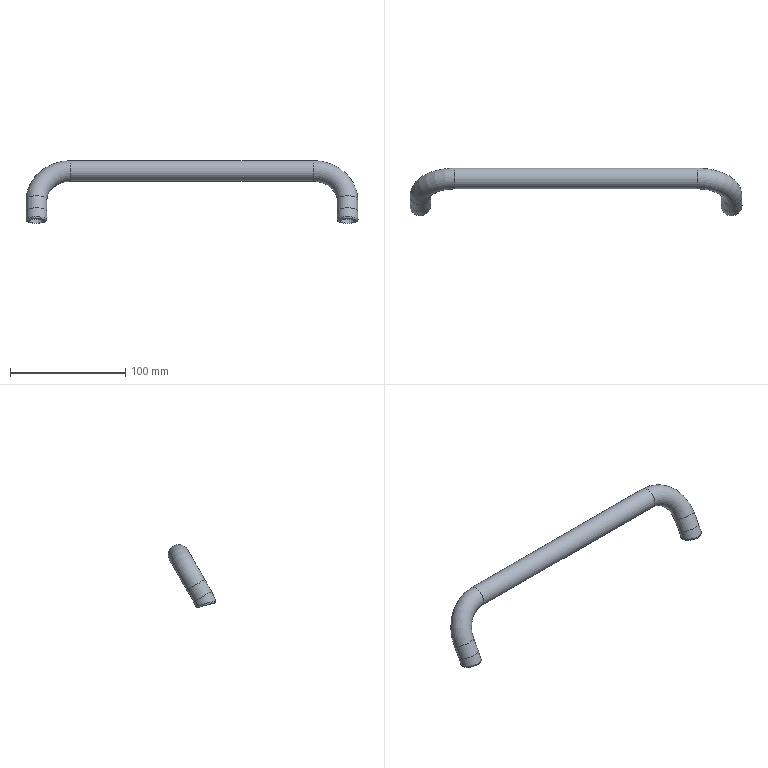Component | NX | FOAM_PAD | 1 solid | 18 faces | box 288 x 41.31 x 54.58 mm | volume 41802 mm3 | torus 8 | cylinder 6 | plane 2 | spline 2 | commonest cylinder face diameters 18 x3 13 x3
STEP:
#1=VALUE_REPRESENTATION_ITEM('',COUNT_MEASURE(0.));
#2=(LENGTH_UNIT()NAMED_UNIT(*)SI_UNIT(.MILLI.,.METRE.));
#3=UNCERTAINTY_MEASURE_WITH_UNIT(LENGTH_MEASURE(0.0508),#2,'','');
#4=(NAMED_UNIT(*)PLANE_ANGLE_UNIT()SI_UNIT($,.RADIAN.));
#5=PLANE_ANGLE_MEASURE_WITH_UNIT(PLANE_ANGLE_MEASURE(0.01745),#4);
#6=DIMENSIONAL_EXPONENTS(0.,0.,0.,0.,0.,0.,0.);
#7=(CONVERSION_BASED_UNIT('',#5)NAMED_UNIT(#6)PLANE_ANGLE_UNIT());
#8=(NAMED_UNIT(*)SI_UNIT($,.STERADIAN.)SOLID_ANGLE_UNIT());
#9=(GEOMETRIC_REPRESENTATION_CONTEXT(3)GLOBAL_UNCERTAINTY_ASSIGNED_CONTEXT((#3))GLOBAL_UNIT_ASSIGNED_CONTEXT((#2,#7,#8))REPRESENTATION_CONTEXT('',''));
#10=REPRESENTATION('',(#1),#9);
#11=VALUE_REPRESENTATION_ITEM('',COUNT_MEASURE(0.));
#12=REPRESENTATION('',(#11),#9);
#13=CARTESIAN_POINT('',(0.,0.,0.));
#14=DIRECTION('',(0.,0.,1.));
#15=DIRECTION('',(1.,0.,0.));
#16=AXIS2_PLACEMENT_3D('',#13,#14,#15);
#17=SHAPE_REPRESENTATION('',(#16),#9);
#18=CARTESIAN_POINT('',(-270.,117.638,-91.446));
#19=VERTEX_POINT('',#18);
#20=CARTESIAN_POINT('',(-272.379,117.638,-91.446));
#21=CARTESIAN_POINT('',(-267.621,117.638,-91.446));
#22=CARTESIAN_POINT('',(-265.309,118.565,-91.699));
#23=CARTESIAN_POINT('',(-261.953,121.809,-92.589));
#24=CARTESIAN_POINT('',(-260.999,124.062,-93.209));
#25=CARTESIAN_POINT('',(-261.001,128.588,-94.462));
#26=CARTESIAN_POINT('',(-261.973,130.853,-95.094));
#27=CARTESIAN_POINT('',(-265.29,134.054,-95.994));
#28=CARTESIAN_POINT('',(-267.615,134.996,-96.263));
#29=CARTESIAN_POINT('',(-272.372,135.,-96.264));
#30=CARTESIAN_POINT('',(-274.703,134.059,-95.996));
#31=CARTESIAN_POINT('',(-278.025,130.858,-95.096));
#32=CARTESIAN_POINT('',(-278.999,128.614,-94.469));
#33=CARTESIAN_POINT('',(-279.001,124.036,-93.202));
#34=CARTESIAN_POINT('',(-278.027,121.79,-92.584));
#35=CARTESIAN_POINT('',(-274.711,118.584,-91.704));
#36=CARTESIAN_POINT('',(-272.379,117.638,-91.446));
#37=CARTESIAN_POINT('',(-267.621,117.638,-91.446));
#38=B_SPLINE_CURVE_WITH_KNOTS('',3,(#20,#21,#22,#23,#24,#25,#26,#27,#28,#29,#30,#31,#32,#33,#34,#35,#36,#37),.UNSPECIFIED.,.T.,.F.,(2,2,2,2,2,2,2,2,2,2,2),(-0.125,0.,0.125,0.25,0.375,0.5,0.625,0.75,0.875,1.,1.125),.UNSPECIFIED.);
#39=EDGE_CURVE('',#19,#19,#38,.T.);
#40=ORIENTED_EDGE('',*,*,#39,.T.);
#41=EDGE_LOOP('',(#40));
#42=FACE_BOUND('',#41,.T.);
#43=CARTESIAN_POINT('',(-270.,121.1,-83.538));
#44=VERTEX_POINT('',#43);
#45=CARTESIAN_POINT('',(-270.,128.894,-88.038));
#46=DIRECTION('',(-0.,-0.5,-0.866));
#47=DIRECTION('',(0.,-0.866,0.5));
#48=AXIS2_PLACEMENT_3D('',#45,#46,#47);
#49=CIRCLE('',#48,9.);
#50=EDGE_CURVE('',#44,#44,#49,.T.);
#51=ORIENTED_EDGE('',*,*,#50,.T.);
#52=EDGE_LOOP('',(#51));
#53=FACE_BOUND('',#52,.T.);
#54=CARTESIAN_POINT('',(-270.,154.875,-103.038));
#55=DIRECTION('',(1.,0.,0.));
#56=DIRECTION('',(0.,0.,-1.));
#57=AXIS2_PLACEMENT_3D('',#54,#55,#56);
#58=TOROIDAL_SURFACE('',#57,30.,9.);
#59=ADVANCED_FACE('',(#42,#53),#58,.T.);
#60=CARTESIAN_POINT('',(-270.,123.265,-84.788));
#61=VERTEX_POINT('',#60);
#62=CARTESIAN_POINT('',(-270.,128.894,-88.038));
#63=DIRECTION('',(-0.,-0.5,-0.866));
#64=DIRECTION('',(0.,-0.866,0.5));
#65=AXIS2_PLACEMENT_3D('',#62,#63,#64);
#66=CIRCLE('',#65,6.5);
#67=EDGE_CURVE('',#61,#61,#66,.T.);
#68=ORIENTED_EDGE('',*,*,#67,.F.);
#69=EDGE_LOOP('',(#68));
#70=FACE_BOUND('',#69,.T.);
#71=CARTESIAN_POINT('',(-270.,119.619,-93.592));
#72=VERTEX_POINT('',#71);
#73=CARTESIAN_POINT('',(-270.,125.897,-95.274));
#74=DIRECTION('',(-0.,-0.2588,-0.9659));
#75=DIRECTION('',(0.,-0.9659,0.2588));
#76=AXIS2_PLACEMENT_3D('',#73,#74,#75);
#77=CIRCLE('',#76,6.5);
#78=EDGE_CURVE('',#72,#72,#77,.T.);
#79=ORIENTED_EDGE('',*,*,#78,.T.);
#80=EDGE_LOOP('',(#79));
#81=FACE_BOUND('',#80,.T.);
#82=CARTESIAN_POINT('',(-270.,154.875,-103.038));
#83=DIRECTION('',(1.,0.,0.));
#84=DIRECTION('',(0.,0.,-1.));
#85=AXIS2_PLACEMENT_3D('',#82,#83,#84);
#86=TOROIDAL_SURFACE('',#85,30.,6.5);
#87=ADVANCED_FACE('',(#70,#81),#86,.F.);
#88=CARTESIAN_POINT('',(-270.,127.081,-73.179));
#89=VERTEX_POINT('',#88);
#90=CARTESIAN_POINT('',(-270.,134.875,-77.679));
#91=DIRECTION('',(-0.,-0.5,-0.866));
#92=DIRECTION('',(0.,-0.866,0.5));
#93=AXIS2_PLACEMENT_3D('',#90,#91,#92);
#94=CIRCLE('',#93,9.);
#95=EDGE_CURVE('',#89,#89,#94,.T.);
#96=ORIENTED_EDGE('',*,*,#95,.T.);
#97=EDGE_LOOP('',(#96));
#98=FACE_BOUND('',#97,.T.);
#99=ORIENTED_EDGE('',*,*,#50,.F.);
#100=EDGE_LOOP('',(#99));
#101=FACE_BOUND('',#100,.T.);
#102=CARTESIAN_POINT('',(-270.,134.875,-77.679));
#103=DIRECTION('',(0.,-0.5,-0.866));
#104=DIRECTION('',(0.,0.866,-0.5));
#105=AXIS2_PLACEMENT_3D('',#102,#103,#104);
#106=CYLINDRICAL_SURFACE('',#105,9.);
#107=ADVANCED_FACE('',(#98,#101),#106,.T.);
#108=CARTESIAN_POINT('',(-270.,129.246,-74.429));
#109=VERTEX_POINT('',#108);
#110=CARTESIAN_POINT('',(-270.,134.875,-77.679));
#111=DIRECTION('',(-0.,-0.5,-0.866));
#112=DIRECTION('',(0.,-0.866,0.5));
#113=AXIS2_PLACEMENT_3D('',#110,#111,#112);
#114=CIRCLE('',#113,6.5);
#115=EDGE_CURVE('',#109,#109,#114,.T.);
#116=ORIENTED_EDGE('',*,*,#115,.F.);
#117=EDGE_LOOP('',(#116));
#118=FACE_BOUND('',#117,.T.);
#119=ORIENTED_EDGE('',*,*,#67,.T.);
#120=EDGE_LOOP('',(#119));
#121=FACE_BOUND('',#120,.T.);
#122=CARTESIAN_POINT('',(-270.,134.875,-77.679));
#123=DIRECTION('',(0.,-0.5,-0.866));
#124=DIRECTION('',(0.,0.866,-0.5));
#125=AXIS2_PLACEMENT_3D('',#122,#123,#124);
#126=CYLINDRICAL_SURFACE('',#125,6.5);
#127=ADVANCED_FACE('',(#118,#121),#126,.F.);
#128=CARTESIAN_POINT('',(-240.,142.081,-47.199));
#129=VERTEX_POINT('',#128);
#130=CARTESIAN_POINT('',(-240.,149.875,-51.699));
#131=DIRECTION('',(-1.,-0.,0.));
#132=DIRECTION('',(0.,-0.866,0.5));
#133=AXIS2_PLACEMENT_3D('',#130,#131,#132);
#134=CIRCLE('',#133,9.);
#135=EDGE_CURVE('',#129,#129,#134,.T.);
#136=ORIENTED_EDGE('',*,*,#135,.T.);
#137=EDGE_LOOP('',(#136));
#138=FACE_BOUND('',#137,.T.);
#139=ORIENTED_EDGE('',*,*,#95,.F.);
#140=EDGE_LOOP('',(#139));
#141=FACE_BOUND('',#140,.T.);
#142=CARTESIAN_POINT('',(-240.,134.875,-77.679));
#143=DIRECTION('',(0.,-0.866,0.5));
#144=DIRECTION('',(0.,-0.5,-0.866));
#145=AXIS2_PLACEMENT_3D('',#142,#143,#144);
#146=TOROIDAL_SURFACE('',#145,30.,9.);
#147=ADVANCED_FACE('',(#138,#141),#146,.T.);
#148=CARTESIAN_POINT('',(-240.,144.246,-48.449));
#149=VERTEX_POINT('',#148);
#150=CARTESIAN_POINT('',(-240.,149.875,-51.699));
#151=DIRECTION('',(-1.,-0.,0.));
#152=DIRECTION('',(0.,-0.866,0.5));
#153=AXIS2_PLACEMENT_3D('',#150,#151,#152);
#154=CIRCLE('',#153,6.5);
#155=EDGE_CURVE('',#149,#149,#154,.T.);
#156=ORIENTED_EDGE('',*,*,#155,.F.);
#157=EDGE_LOOP('',(#156));
#158=FACE_BOUND('',#157,.T.);
#159=ORIENTED_EDGE('',*,*,#115,.T.);
#160=EDGE_LOOP('',(#159));
#161=FACE_BOUND('',#160,.T.);
#162=CARTESIAN_POINT('',(-240.,134.875,-77.679));
#163=DIRECTION('',(0.,-0.866,0.5));
#164=DIRECTION('',(0.,-0.5,-0.866));
#165=AXIS2_PLACEMENT_3D('',#162,#163,#164);
#166=TOROIDAL_SURFACE('',#165,30.,6.5);
#167=ADVANCED_FACE('',(#158,#161),#166,.F.);
#168=CARTESIAN_POINT('',(-30.,142.081,-47.199));
#169=VERTEX_POINT('',#168);
#170=CARTESIAN_POINT('',(-30.,149.875,-51.699));
#171=DIRECTION('',(-1.,-0.,0.));
#172=DIRECTION('',(0.,-0.866,0.5));
#173=AXIS2_PLACEMENT_3D('',#170,#171,#172);
#174=CIRCLE('',#173,9.);
#175=EDGE_CURVE('',#169,#169,#174,.T.);
#176=ORIENTED_EDGE('',*,*,#175,.T.);
#177=EDGE_LOOP('',(#176));
#178=FACE_BOUND('',#177,.T.);
#179=ORIENTED_EDGE('',*,*,#135,.F.);
#180=EDGE_LOOP('',(#179));
#181=FACE_BOUND('',#180,.T.);
#182=CARTESIAN_POINT('',(-30.,149.875,-51.699));
#183=DIRECTION('',(-1.,0.,0.));
#184=DIRECTION('',(0.,0.,1.));
#185=AXIS2_PLACEMENT_3D('',#182,#183,#184);
#186=CYLINDRICAL_SURFACE('',#185,9.);
#187=ADVANCED_FACE('',(#178,#181),#186,.T.);
#188=CARTESIAN_POINT('',(-30.,144.246,-48.449));
#189=VERTEX_POINT('',#188);
#190=CARTESIAN_POINT('',(-30.,149.875,-51.699));
#191=DIRECTION('',(-1.,-0.,0.));
#192=DIRECTION('',(0.,-0.866,0.5));
#193=AXIS2_PLACEMENT_3D('',#190,#191,#192);
#194=CIRCLE('',#193,6.5);
#195=EDGE_CURVE('',#189,#189,#194,.T.);
#196=ORIENTED_EDGE('',*,*,#195,.F.);
#197=EDGE_LOOP('',(#196));
#198=FACE_BOUND('',#197,.T.);
#199=ORIENTED_EDGE('',*,*,#155,.T.);
#200=EDGE_LOOP('',(#199));
#201=FACE_BOUND('',#200,.T.);
#202=CARTESIAN_POINT('',(-30.,149.875,-51.699));
#203=DIRECTION('',(-1.,0.,0.));
#204=DIRECTION('',(0.,0.,1.));
#205=AXIS2_PLACEMENT_3D('',#202,#203,#204);
#206=CYLINDRICAL_SURFACE('',#205,6.5);
#207=ADVANCED_FACE('',(#198,#201),#206,.F.);
#208=CARTESIAN_POINT('',(-0.,127.081,-73.179));
#209=VERTEX_POINT('',#208);
#210=CARTESIAN_POINT('',(-0.,134.875,-77.679));
#211=DIRECTION('',(0.,0.5,0.866));
#212=DIRECTION('',(0.,-0.866,0.5));
#213=AXIS2_PLACEMENT_3D('',#210,#211,#212);
#214=CIRCLE('',#213,9.);
#215=EDGE_CURVE('',#209,#209,#214,.T.);
#216=ORIENTED_EDGE('',*,*,#215,.T.);
#217=EDGE_LOOP('',(#216));
#218=FACE_BOUND('',#217,.T.);
#219=ORIENTED_EDGE('',*,*,#175,.F.);
#220=EDGE_LOOP('',(#219));
#221=FACE_BOUND('',#220,.T.);
#222=CARTESIAN_POINT('',(-30.,134.875,-77.679));
#223=DIRECTION('',(0.,-0.866,0.5));
#224=DIRECTION('',(0.,-0.5,-0.866));
#225=AXIS2_PLACEMENT_3D('',#222,#223,#224);
#226=TOROIDAL_SURFACE('',#225,30.,9.);
#227=ADVANCED_FACE('',(#218,#221),#226,.T.);
#228=CARTESIAN_POINT('',(-0.,129.246,-74.429));
#229=VERTEX_POINT('',#228);
#230=CARTESIAN_POINT('',(-0.,134.875,-77.679));
#231=DIRECTION('',(0.,0.5,0.866));
#232=DIRECTION('',(0.,-0.866,0.5));
#233=AXIS2_PLACEMENT_3D('',#230,#231,#232);
#234=CIRCLE('',#233,6.5);
#235=EDGE_CURVE('',#229,#229,#234,.T.);
#236=ORIENTED_EDGE('',*,*,#235,.F.);
#237=EDGE_LOOP('',(#236));
#238=FACE_BOUND('',#237,.T.);
#239=ORIENTED_EDGE('',*,*,#195,.T.);
#240=EDGE_LOOP('',(#239));
#241=FACE_BOUND('',#240,.T.);
#242=CARTESIAN_POINT('',(-30.,134.875,-77.679));
#243=DIRECTION('',(0.,-0.866,0.5));
#244=DIRECTION('',(0.,-0.5,-0.866));
#245=AXIS2_PLACEMENT_3D('',#242,#243,#244);
#246=TOROIDAL_SURFACE('',#245,30.,6.5);
#247=ADVANCED_FACE('',(#238,#241),#246,.F.);
#248=CARTESIAN_POINT('',(-0.,121.1,-83.538));
#249=VERTEX_POINT('',#248);
#250=CARTESIAN_POINT('',(-0.,128.894,-88.038));
#251=DIRECTION('',(0.,0.5,0.866));
#252=DIRECTION('',(0.,-0.866,0.5));
#253=AXIS2_PLACEMENT_3D('',#250,#251,#252);
#254=CIRCLE('',#253,9.);
#255=EDGE_CURVE('',#249,#249,#254,.T.);
#256=ORIENTED_EDGE('',*,*,#255,.T.);
#257=EDGE_LOOP('',(#256));
#258=FACE_BOUND('',#257,.T.);
#259=ORIENTED_EDGE('',*,*,#215,.F.);
#260=EDGE_LOOP('',(#259));
#261=FACE_BOUND('',#260,.T.);
#262=CARTESIAN_POINT('',(-0.,128.894,-88.038));
#263=DIRECTION('',(0.,0.5,0.866));
#264=DIRECTION('',(0.,-0.866,0.5));
#265=AXIS2_PLACEMENT_3D('',#262,#263,#264);
#266=CYLINDRICAL_SURFACE('',#265,9.);
#267=ADVANCED_FACE('',(#258,#261),#266,.T.);
#268=CARTESIAN_POINT('',(-0.,123.265,-84.788));
#269=VERTEX_POINT('',#268);
#270=CARTESIAN_POINT('',(-0.,128.894,-88.038));
#271=DIRECTION('',(0.,0.5,0.866));
#272=DIRECTION('',(0.,-0.866,0.5));
#273=AXIS2_PLACEMENT_3D('',#270,#271,#272);
#274=CIRCLE('',#273,6.5);
#275=EDGE_CURVE('',#269,#269,#274,.T.);
#276=ORIENTED_EDGE('',*,*,#275,.F.);
#277=EDGE_LOOP('',(#276));
#278=FACE_BOUND('',#277,.T.);
#279=ORIENTED_EDGE('',*,*,#235,.T.);
#280=EDGE_LOOP('',(#279));
#281=FACE_BOUND('',#280,.T.);
#282=CARTESIAN_POINT('',(-0.,128.894,-88.038));
#283=DIRECTION('',(0.,0.5,0.866));
#284=DIRECTION('',(0.,-0.866,0.5));
#285=AXIS2_PLACEMENT_3D('',#282,#283,#284);
#286=CYLINDRICAL_SURFACE('',#285,6.5);
#287=ADVANCED_FACE('',(#278,#281),#286,.F.);
#288=ORIENTED_EDGE('',*,*,#275,.T.);
#289=EDGE_LOOP('',(#288));
#290=FACE_BOUND('',#289,.T.);
#291=CARTESIAN_POINT('',(-0.,119.619,-93.592));
#292=VERTEX_POINT('',#291);
#293=CARTESIAN_POINT('',(-0.,125.897,-95.274));
#294=DIRECTION('',(0.,0.2588,0.9659));
#295=DIRECTION('',(0.,-0.9659,0.2588));
#296=AXIS2_PLACEMENT_3D('',#293,#294,#295);
#297=CIRCLE('',#296,6.5);
#298=EDGE_CURVE('',#292,#292,#297,.T.);
#299=ORIENTED_EDGE('',*,*,#298,.F.);
#300=EDGE_LOOP('',(#299));
#301=FACE_BOUND('',#300,.T.);
#302=CARTESIAN_POINT('',(-0.,154.875,-103.038));
#303=DIRECTION('',(1.,0.,0.));
#304=DIRECTION('',(0.,0.,-1.));
#305=AXIS2_PLACEMENT_3D('',#302,#303,#304);
#306=TOROIDAL_SURFACE('',#305,30.,6.5);
#307=ADVANCED_FACE('',(#290,#301),#306,.F.);
#308=CARTESIAN_POINT('',(-0.,117.638,-91.446));
#309=VERTEX_POINT('',#308);
#310=CARTESIAN_POINT('',(-2.379,117.638,-91.446));
#311=CARTESIAN_POINT('',(2.379,117.638,-91.446));
#312=CARTESIAN_POINT('',(4.711,118.584,-91.704));
#313=CARTESIAN_POINT('',(8.027,121.79,-92.584));
#314=CARTESIAN_POINT('',(9.001,124.036,-93.202));
#315=CARTESIAN_POINT('',(8.999,128.614,-94.469));
#316=CARTESIAN_POINT('',(8.025,130.858,-95.096));
#317=CARTESIAN_POINT('',(4.703,134.059,-95.996));
#318=CARTESIAN_POINT('',(2.372,135.,-96.264));
#319=CARTESIAN_POINT('',(-2.385,134.996,-96.263));
#320=CARTESIAN_POINT('',(-4.71,134.054,-95.994));
#321=CARTESIAN_POINT('',(-8.027,130.853,-95.094));
#322=CARTESIAN_POINT('',(-8.999,128.588,-94.462));
#323=CARTESIAN_POINT('',(-9.001,124.062,-93.209));
#324=CARTESIAN_POINT('',(-8.047,121.809,-92.589));
#325=CARTESIAN_POINT('',(-4.691,118.565,-91.699));
#326=CARTESIAN_POINT('',(-2.379,117.638,-91.446));
#327=CARTESIAN_POINT('',(2.379,117.638,-91.446));
#328=B_SPLINE_CURVE_WITH_KNOTS('',3,(#310,#311,#312,#313,#314,#315,#316,#317,#318,#319,#320,#321,#322,#323,#324,#325,#326,#327),.UNSPECIFIED.,.T.,.F.,(2,2,2,2,2,2,2,2,2,2,2),(-0.125,0.,0.125,0.25,0.375,0.5,0.625,0.75,0.875,1.,1.125),.UNSPECIFIED.);
#329=EDGE_CURVE('',#309,#309,#328,.T.);
#330=ORIENTED_EDGE('',*,*,#329,.T.);
#331=EDGE_LOOP('',(#330));
#332=FACE_BOUND('',#331,.T.);
#333=ORIENTED_EDGE('',*,*,#255,.F.);
#334=EDGE_LOOP('',(#333));
#335=FACE_BOUND('',#334,.T.);
#336=CARTESIAN_POINT('',(-0.,154.875,-103.038));
#337=DIRECTION('',(1.,0.,0.));
#338=DIRECTION('',(0.,0.,-1.));
#339=AXIS2_PLACEMENT_3D('',#336,#337,#338);
#340=TOROIDAL_SURFACE('',#339,30.,9.);
#341=ADVANCED_FACE('',(#332,#335),#340,.T.);
#342=CARTESIAN_POINT('',(-270.,118.682,-93.341));
#343=VERTEX_POINT('',#342);
#344=CARTESIAN_POINT('',(-268.017,118.682,-93.341));
#345=CARTESIAN_POINT('',(-271.983,118.682,-93.341));
#346=CARTESIAN_POINT('',(-273.927,119.472,-93.552));
#347=CARTESIAN_POINT('',(-276.69,122.149,-94.269));
#348=CARTESIAN_POINT('',(-277.501,124.025,-94.772));
#349=CARTESIAN_POINT('',(-277.499,127.849,-95.797));
#350=CARTESIAN_POINT('',(-276.687,129.725,-96.299));
#351=CARTESIAN_POINT('',(-273.919,132.403,-97.017));
#352=CARTESIAN_POINT('',(-271.977,133.192,-97.228));
#353=CARTESIAN_POINT('',(-268.012,133.189,-97.228));
#354=CARTESIAN_POINT('',(-266.074,132.399,-97.016));
#355=CARTESIAN_POINT('',(-263.311,129.72,-96.298));
#356=CARTESIAN_POINT('',(-262.501,127.828,-95.791));
#357=CARTESIAN_POINT('',(-262.499,124.047,-94.778));
#358=CARTESIAN_POINT('',(-263.293,122.165,-94.274));
#359=CARTESIAN_POINT('',(-266.09,119.456,-93.548));
#360=CARTESIAN_POINT('',(-268.017,118.682,-93.341));
#361=CARTESIAN_POINT('',(-271.983,118.682,-93.341));
#362=B_SPLINE_CURVE_WITH_KNOTS('',3,(#344,#345,#346,#347,#348,#349,#350,#351,#352,#353,#354,#355,#356,#357,#358,#359,#360,#361),.UNSPECIFIED.,.T.,.F.,(2,2,2,2,2,2,2,2,2,2,2),(-0.125,0.,0.125,0.25,0.375,0.5,0.625,0.75,0.875,1.,1.125),.UNSPECIFIED.);
#363=EDGE_CURVE('',#343,#343,#362,.T.);
#364=ORIENTED_EDGE('',*,*,#363,.T.);
#365=EDGE_LOOP('',(#364));
#366=FACE_BOUND('',#365,.T.);
#367=ORIENTED_EDGE('',*,*,#78,.F.);
#368=EDGE_LOOP('',(#367));
#369=FACE_BOUND('',#368,.T.);
#370=CARTESIAN_POINT('',(-270.,125.897,-95.274));
#371=DIRECTION('',(-0.,-0.2588,-0.9659));
#372=DIRECTION('',(0.,-0.9659,0.2588));
#373=AXIS2_PLACEMENT_3D('',#370,#371,#372);
#374=PLANE('',#373);
#375=ADVANCED_FACE('',(#366,#369),#374,.T.);
#376=CARTESIAN_POINT('',(-0.,118.682,-93.341));
#377=VERTEX_POINT('',#376);
#378=CARTESIAN_POINT('',(1.983,118.682,-93.341));
#379=CARTESIAN_POINT('',(-1.983,118.682,-93.341));
#380=CARTESIAN_POINT('',(-3.91,119.456,-93.548));
#381=CARTESIAN_POINT('',(-6.707,122.165,-94.274));
#382=CARTESIAN_POINT('',(-7.501,124.047,-94.778));
#383=CARTESIAN_POINT('',(-7.499,127.828,-95.791));
#384=CARTESIAN_POINT('',(-6.689,129.72,-96.298));
#385=CARTESIAN_POINT('',(-3.926,132.399,-97.016));
#386=CARTESIAN_POINT('',(-1.988,133.189,-97.228));
#387=CARTESIAN_POINT('',(1.977,133.192,-97.228));
#388=CARTESIAN_POINT('',(3.92,132.403,-97.017));
#389=CARTESIAN_POINT('',(6.687,129.725,-96.299));
#390=CARTESIAN_POINT('',(7.499,127.849,-95.797));
#391=CARTESIAN_POINT('',(7.501,124.025,-94.772));
#392=CARTESIAN_POINT('',(6.69,122.149,-94.269));
#393=CARTESIAN_POINT('',(3.927,119.472,-93.552));
#394=CARTESIAN_POINT('',(1.983,118.682,-93.341));
#395=CARTESIAN_POINT('',(-1.983,118.682,-93.341));
#396=B_SPLINE_CURVE_WITH_KNOTS('',3,(#378,#379,#380,#381,#382,#383,#384,#385,#386,#387,#388,#389,#390,#391,#392,#393,#394,#395),.UNSPECIFIED.,.T.,.F.,(2,2,2,2,2,2,2,2,2,2,2),(-0.125,0.,0.125,0.25,0.375,0.5,0.625,0.75,0.875,1.,1.125),.UNSPECIFIED.);
#397=EDGE_CURVE('',#377,#377,#396,.T.);
#398=ORIENTED_EDGE('',*,*,#397,.T.);
#399=EDGE_LOOP('',(#398));
#400=FACE_BOUND('',#399,.T.);
#401=ORIENTED_EDGE('',*,*,#298,.T.);
#402=EDGE_LOOP('',(#401));
#403=FACE_BOUND('',#402,.T.);
#404=CARTESIAN_POINT('',(-0.,125.897,-95.274));
#405=DIRECTION('',(0.,0.2588,0.9659));
#406=DIRECTION('',(0.,-0.9659,0.2588));
#407=AXIS2_PLACEMENT_3D('',#404,#405,#406);
#408=PLANE('',#407);
#409=ADVANCED_FACE('',(#400,#403),#408,.F.);
#410=ORIENTED_EDGE('',*,*,#39,.F.);
#411=EDGE_LOOP('',(#410));
#412=FACE_BOUND('',#411,.T.);
#413=ORIENTED_EDGE('',*,*,#363,.F.);
#414=EDGE_LOOP('',(#413));
#415=FACE_BOUND('',#414,.T.);
#416=CARTESIAN_POINT('',(-269.053,117.686,-91.459));
#417=CARTESIAN_POINT('',(-269.047,117.223,-92.95));
#418=CARTESIAN_POINT('',(-269.211,118.722,-93.351));
#419=CARTESIAN_POINT('',(-270.237,117.565,-91.426));
#420=CARTESIAN_POINT('',(-270.239,117.1,-92.917));
#421=CARTESIAN_POINT('',(-270.197,118.621,-93.324));
#422=CARTESIAN_POINT('',(-271.423,117.672,-91.455));
#423=CARTESIAN_POINT('',(-271.432,117.208,-92.946));
#424=CARTESIAN_POINT('',(-271.186,118.71,-93.348));
#425=CARTESIAN_POINT('',(-273.687,118.319,-91.632));
#426=CARTESIAN_POINT('',(-273.71,117.864,-93.121));
#427=CARTESIAN_POINT('',(-273.072,119.25,-93.493));
#428=CARTESIAN_POINT('',(-274.75,118.86,-91.78));
#429=CARTESIAN_POINT('',(-274.778,118.411,-93.268));
#430=CARTESIAN_POINT('',(-273.959,119.702,-93.614));
#431=CARTESIAN_POINT('',(-277.489,120.999,-92.367));
#432=CARTESIAN_POINT('',(-277.52,120.574,-93.847));
#433=CARTESIAN_POINT('',(-276.241,121.488,-94.092));
#434=CARTESIAN_POINT('',(-278.703,123.156,-92.959));
#435=CARTESIAN_POINT('',(-278.727,122.742,-94.429));
#436=CARTESIAN_POINT('',(-277.252,123.289,-94.575));
#437=CARTESIAN_POINT('',(-279.074,126.533,-93.893));
#438=CARTESIAN_POINT('',(-279.072,126.143,-95.34));
#439=CARTESIAN_POINT('',(-277.561,126.11,-95.331));
#440=CARTESIAN_POINT('',(-278.966,127.687,-94.213));
#441=CARTESIAN_POINT('',(-278.955,127.298,-95.649));
#442=CARTESIAN_POINT('',(-277.471,127.074,-95.589));
#443=CARTESIAN_POINT('',(-278.299,129.867,-94.82));
#444=CARTESIAN_POINT('',(-278.269,129.472,-96.232));
#445=CARTESIAN_POINT('',(-276.916,128.897,-96.078));
#446=CARTESIAN_POINT('',(-277.748,130.884,-95.104));
#447=CARTESIAN_POINT('',(-277.712,130.483,-96.503));
#448=CARTESIAN_POINT('',(-276.456,129.747,-96.306));
#449=CARTESIAN_POINT('',(-275.509,133.556,-95.853));
#450=CARTESIAN_POINT('',(-275.471,133.12,-97.209));
#451=CARTESIAN_POINT('',(-274.591,131.982,-96.904));
#452=CARTESIAN_POINT('',(-273.3,134.71,-96.181));
#453=CARTESIAN_POINT('',(-273.269,134.263,-97.515));
#454=CARTESIAN_POINT('',(-272.75,132.949,-97.163));
#455=CARTESIAN_POINT('',(-268.593,135.19,-96.317));
#456=CARTESIAN_POINT('',(-268.61,134.733,-97.641));
#457=CARTESIAN_POINT('',(-268.827,133.351,-97.271));
#458=CARTESIAN_POINT('',(-266.18,134.505,-96.122));
#459=CARTESIAN_POINT('',(-266.209,134.056,-97.46));
#460=CARTESIAN_POINT('',(-266.817,132.777,-97.117));
#461=CARTESIAN_POINT('',(-263.412,132.344,-95.513));
#462=CARTESIAN_POINT('',(-263.454,131.93,-96.89));
#463=CARTESIAN_POINT('',(-264.51,130.968,-96.633));
#464=CARTESIAN_POINT('',(-262.652,131.46,-95.265));
#465=CARTESIAN_POINT('',(-262.691,131.054,-96.656));
#466=CARTESIAN_POINT('',(-263.876,130.229,-96.434));
#467=CARTESIAN_POINT('',(-261.528,129.463,-94.707));
#468=CARTESIAN_POINT('',(-261.554,129.07,-96.124));
#469=CARTESIAN_POINT('',(-262.94,128.559,-95.987));
#470=CARTESIAN_POINT('',(-261.172,128.356,-94.399));
#471=CARTESIAN_POINT('',(-261.19,127.966,-95.828));
#472=CARTESIAN_POINT('',(-262.644,127.633,-95.739));
#473=CARTESIAN_POINT('',(-260.804,124.98,-93.462));
#474=CARTESIAN_POINT('',(-260.79,124.577,-94.92));
#475=CARTESIAN_POINT('',(-262.337,124.813,-94.983));
#476=CARTESIAN_POINT('',(-261.524,122.627,-92.814));
#477=CARTESIAN_POINT('',(-261.499,122.215,-94.287));
#478=CARTESIAN_POINT('',(-262.936,122.847,-94.457));
#479=CARTESIAN_POINT('',(-263.738,119.983,-92.088));
#480=CARTESIAN_POINT('',(-263.705,119.548,-93.573));
#481=CARTESIAN_POINT('',(-264.781,120.64,-93.865));
#482=CARTESIAN_POINT('',(-264.66,119.24,-91.884));
#483=CARTESIAN_POINT('',(-264.63,118.796,-93.371));
#484=CARTESIAN_POINT('',(-265.55,120.019,-93.699));
#485=CARTESIAN_POINT('',(-266.734,118.15,-91.586));
#486=CARTESIAN_POINT('',(-266.713,117.693,-93.076));
#487=CARTESIAN_POINT('',(-267.278,119.11,-93.455));
#488=CARTESIAN_POINT('',(-267.87,117.807,-91.492));
#489=CARTESIAN_POINT('',(-267.856,117.345,-92.982));
#490=CARTESIAN_POINT('',(-268.225,118.823,-93.378));
#491=CARTESIAN_POINT('',(-269.053,117.686,-91.459));
#492=CARTESIAN_POINT('',(-269.047,117.223,-92.95));
#493=CARTESIAN_POINT('',(-269.211,118.722,-93.351));
#494=(BOUNDED_SURFACE()B_SPLINE_SURFACE(3,2,((#416,#417,#418),(#419,#420,#421),(#422,#423,#424),(#425,#426,#427),(#428,#429,#430),(#431,#432,#433),(#434,#435,#436),(#437,#438,#439),(#440,#441,#442),(#443,#444,#445),(#446,#447,#448),(#449,#450,#451),(#452,#453,#454),(#455,#456,#457),(#458,#459,#460),(#461,#462,#463),(#464,#465,#466),(#467,#468,#469),(#470,#471,#472),(#473,#474,#475),(#476,#477,#478),(#479,#480,#481),(#482,#483,#484),(#485,#486,#487),(#488,#489,#490),(#491,#492,#493)),.UNSPECIFIED.,.T.,.F.,.F.)B_SPLINE_SURFACE_WITH_KNOTS((1,3,2,2,2,2,2,2,2,2,2,2,2,3,1),(3,3),(-0.0625,0.,0.0625,0.125,0.25,0.3125,0.375,0.5,0.625,0.6875,0.75,0.875,0.9375,1.,1.062),(0.,1.),.UNSPECIFIED.)GEOMETRIC_REPRESENTATION_ITEM()RATIONAL_B_SPLINE_SURFACE(((1.,0.6929,1.),(1.,0.6927,1.),(1.,0.6929,1.),(1.,0.6937,1.),(1.,0.6945,1.),(1.,0.6976,1.),(1.,0.7009,1.),(1.,0.7075,1.),(1.,0.7099,1.),(1.,0.715,1.),(1.,0.7177,1.),(1.,0.7252,1.),(1.,0.7293,1.),(1.,0.731,1.),(1.,0.7284,1.),(1.,0.7217,1.),(1.,0.7192,1.),(1.,0.714,1.),(1.,0.7114,1.),(1.,0.7042,1.),(1.,0.7002,1.),(1.,0.6961,1.),(1.,0.695,1.),(1.,0.6935,1.),(1.,0.693,1.),(1.,0.6929,1.)))REPRESENTATION_ITEM('')SURFACE());
#495=ADVANCED_FACE('',(#412,#415),#494,.T.);
#496=ORIENTED_EDGE('',*,*,#397,.F.);
#497=EDGE_LOOP('',(#496));
#498=FACE_BOUND('',#497,.T.);
#499=ORIENTED_EDGE('',*,*,#329,.F.);
#500=EDGE_LOOP('',(#499));
#501=FACE_BOUND('',#500,.T.);
#502=CARTESIAN_POINT('',(-0.7888,118.722,-93.351));
#503=CARTESIAN_POINT('',(-0.9531,117.223,-92.95));
#504=CARTESIAN_POINT('',(-0.9465,117.686,-91.459));
#505=CARTESIAN_POINT('',(0.1973,118.621,-93.324));
#506=CARTESIAN_POINT('',(0.2387,117.1,-92.917));
#507=CARTESIAN_POINT('',(0.2368,117.565,-91.426));
#508=CARTESIAN_POINT('',(1.186,118.71,-93.348));
#509=CARTESIAN_POINT('',(1.432,117.208,-92.946));
#510=CARTESIAN_POINT('',(1.423,117.672,-91.455));
#511=CARTESIAN_POINT('',(3.072,119.25,-93.493));
#512=CARTESIAN_POINT('',(3.71,117.864,-93.121));
#513=CARTESIAN_POINT('',(3.687,118.319,-91.632));
#514=CARTESIAN_POINT('',(3.959,119.702,-93.614));
#515=CARTESIAN_POINT('',(4.778,118.411,-93.268));
#516=CARTESIAN_POINT('',(4.75,118.86,-91.78));
#517=CARTESIAN_POINT('',(6.241,121.488,-94.092));
#518=CARTESIAN_POINT('',(7.52,120.574,-93.847));
#519=CARTESIAN_POINT('',(7.489,120.999,-92.367));
#520=CARTESIAN_POINT('',(7.252,123.289,-94.575));
#521=CARTESIAN_POINT('',(8.727,122.742,-94.429));
#522=CARTESIAN_POINT('',(8.703,123.156,-92.959));
#523=CARTESIAN_POINT('',(7.561,126.11,-95.331));
#524=CARTESIAN_POINT('',(9.072,126.143,-95.34));
#525=CARTESIAN_POINT('',(9.074,126.533,-93.893));
#526=CARTESIAN_POINT('',(7.471,127.074,-95.589));
#527=CARTESIAN_POINT('',(8.955,127.298,-95.649));
#528=CARTESIAN_POINT('',(8.966,127.687,-94.213));
#529=CARTESIAN_POINT('',(6.916,128.897,-96.078));
#530=CARTESIAN_POINT('',(8.269,129.472,-96.232));
#531=CARTESIAN_POINT('',(8.299,129.867,-94.82));
#532=CARTESIAN_POINT('',(6.456,129.747,-96.306));
#533=CARTESIAN_POINT('',(7.712,130.483,-96.503));
#534=CARTESIAN_POINT('',(7.748,130.884,-95.104));
#535=CARTESIAN_POINT('',(4.591,131.982,-96.904));
#536=CARTESIAN_POINT('',(5.471,133.12,-97.209));
#537=CARTESIAN_POINT('',(5.509,133.556,-95.853));
#538=CARTESIAN_POINT('',(2.75,132.949,-97.163));
#539=CARTESIAN_POINT('',(3.269,134.263,-97.515));
#540=CARTESIAN_POINT('',(3.3,134.71,-96.181));
#541=CARTESIAN_POINT('',(-1.173,133.351,-97.271));
#542=CARTESIAN_POINT('',(-1.39,134.733,-97.641));
#543=CARTESIAN_POINT('',(-1.407,135.19,-96.317));
#544=CARTESIAN_POINT('',(-3.183,132.777,-97.117));
#545=CARTESIAN_POINT('',(-3.791,134.056,-97.46));
#546=CARTESIAN_POINT('',(-3.82,134.505,-96.122));
#547=CARTESIAN_POINT('',(-5.49,130.968,-96.633));
#548=CARTESIAN_POINT('',(-6.546,131.93,-96.89));
#549=CARTESIAN_POINT('',(-6.588,132.344,-95.513));
#550=CARTESIAN_POINT('',(-6.124,130.229,-96.434));
#551=CARTESIAN_POINT('',(-7.309,131.054,-96.656));
#552=CARTESIAN_POINT('',(-7.348,131.46,-95.265));
#553=CARTESIAN_POINT('',(-7.06,128.559,-95.987));
#554=CARTESIAN_POINT('',(-8.446,129.07,-96.124));
#555=CARTESIAN_POINT('',(-8.472,129.463,-94.707));
#556=CARTESIAN_POINT('',(-7.356,127.633,-95.739));
#557=CARTESIAN_POINT('',(-8.81,127.966,-95.828));
#558=CARTESIAN_POINT('',(-8.828,128.356,-94.399));
#559=CARTESIAN_POINT('',(-7.663,124.813,-94.983));
#560=CARTESIAN_POINT('',(-9.21,124.577,-94.92));
#561=CARTESIAN_POINT('',(-9.196,124.98,-93.462));
#562=CARTESIAN_POINT('',(-7.064,122.847,-94.457));
#563=CARTESIAN_POINT('',(-8.501,122.215,-94.287));
#564=CARTESIAN_POINT('',(-8.476,122.627,-92.814));
#565=CARTESIAN_POINT('',(-5.219,120.64,-93.865));
#566=CARTESIAN_POINT('',(-6.295,119.548,-93.573));
#567=CARTESIAN_POINT('',(-6.262,119.983,-92.088));
#568=CARTESIAN_POINT('',(-4.45,120.019,-93.699));
#569=CARTESIAN_POINT('',(-5.37,118.796,-93.371));
#570=CARTESIAN_POINT('',(-5.34,119.24,-91.884));
#571=CARTESIAN_POINT('',(-2.722,119.11,-93.455));
#572=CARTESIAN_POINT('',(-3.287,117.693,-93.076));
#573=CARTESIAN_POINT('',(-3.266,118.15,-91.586));
#574=CARTESIAN_POINT('',(-1.775,118.823,-93.378));
#575=CARTESIAN_POINT('',(-2.144,117.345,-92.982));
#576=CARTESIAN_POINT('',(-2.13,117.807,-91.492));
#577=CARTESIAN_POINT('',(-0.7888,118.722,-93.351));
#578=CARTESIAN_POINT('',(-0.9531,117.223,-92.95));
#579=CARTESIAN_POINT('',(-0.9465,117.686,-91.459));
#580=(BOUNDED_SURFACE()B_SPLINE_SURFACE(3,2,((#502,#503,#504),(#505,#506,#507),(#508,#509,#510),(#511,#512,#513),(#514,#515,#516),(#517,#518,#519),(#520,#521,#522),(#523,#524,#525),(#526,#527,#528),(#529,#530,#531),(#532,#533,#534),(#535,#536,#537),(#538,#539,#540),(#541,#542,#543),(#544,#545,#546),(#547,#548,#549),(#550,#551,#552),(#553,#554,#555),(#556,#557,#558),(#559,#560,#561),(#562,#563,#564),(#565,#566,#567),(#568,#569,#570),(#571,#572,#573),(#574,#575,#576),(#577,#578,#579)),.UNSPECIFIED.,.T.,.F.,.F.)B_SPLINE_SURFACE_WITH_KNOTS((1,3,2,2,2,2,2,2,2,2,2,2,2,3,1),(3,3),(-0.0625,0.,0.0625,0.125,0.25,0.3125,0.375,0.5,0.625,0.6875,0.75,0.875,0.9375,1.,1.062),(0.,1.),.UNSPECIFIED.)GEOMETRIC_REPRESENTATION_ITEM()RATIONAL_B_SPLINE_SURFACE(((1.,0.6929,1.),(1.,0.6927,1.),(1.,0.6929,1.),(1.,0.6937,1.),(1.,0.6945,1.),(1.,0.6976,1.),(1.,0.7009,1.),(1.,0.7075,1.),(1.,0.7099,1.),(1.,0.715,1.),(1.,0.7177,1.),(1.,0.7252,1.),(1.,0.7293,1.),(1.,0.731,1.),(1.,0.7284,1.),(1.,0.7217,1.),(1.,0.7192,1.),(1.,0.714,1.),(1.,0.7114,1.),(1.,0.7042,1.),(1.,0.7002,1.),(1.,0.6961,1.),(1.,0.695,1.),(1.,0.6935,1.),(1.,0.693,1.),(1.,0.6929,1.)))REPRESENTATION_ITEM('')SURFACE());
#581=ADVANCED_FACE('',(#498,#501),#580,.T.);
#582=CLOSED_SHELL('',(#59,#87,#107,#127,#147,#167,#187,#207,#227,#247,#267,#287,#307,#341,#375,#409,#495,#581));
#583=MANIFOLD_SOLID_BREP('',#582);
#584=ADVANCED_BREP_SHAPE_REPRESENTATION('',(#583),#9);
#585=SHAPE_REPRESENTATION_RELATIONSHIP('','',#17,#584);
#586=PRESENTATION_LAYER_ASSIGNMENT('','',(#583));
#587=COLOUR_RGB('',1.,0.6,0.);
#588=FILL_AREA_STYLE_COLOUR('',#587);
#589=FILL_AREA_STYLE('',(#588));
#590=SURFACE_STYLE_FILL_AREA(#589);
#591=SURFACE_SIDE_STYLE('',(#590));
#592=SURFACE_STYLE_USAGE(.BOTH.,#591);
#593=PRESENTATION_STYLE_ASSIGNMENT((#592));
#594=STYLED_ITEM('',(#593),#583);
#595=MECHANICAL_DESIGN_GEOMETRIC_PRESENTATION_REPRESENTATION('',(#594),#9);